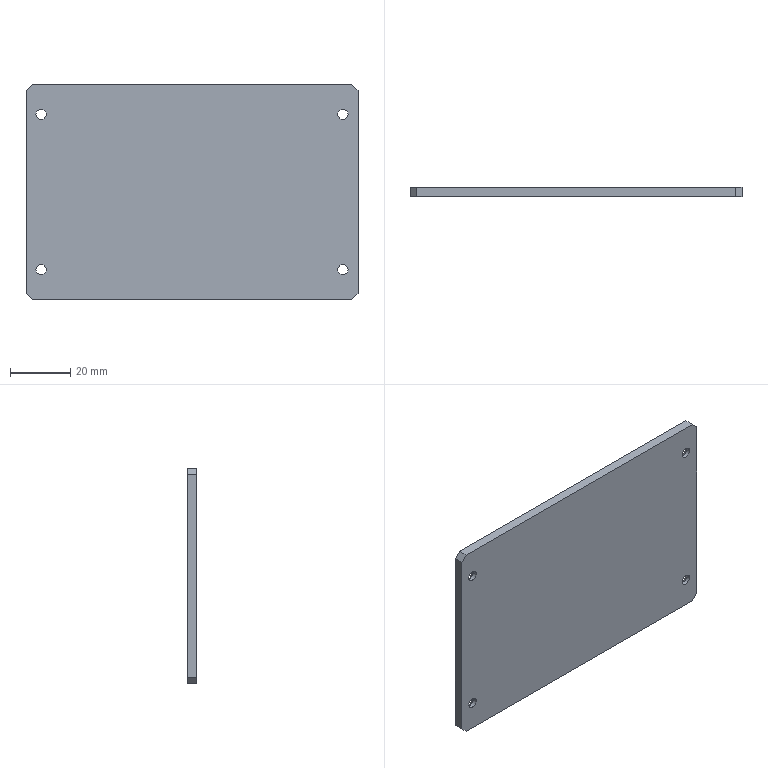Component | SolidWorks | 170423A4-SafetyPowerProbeFixingPlate5-1 | 1 solid | 26 faces | box 110 x 3 x 71.5 mm | volume 23384 mm3 | plane 10 | cone 8 | cylinder 8 | commonest cylinder face diameters 3.4 x8
build123d program:
from build123d import *

# Parameters (mm, degrees)
SKETCH1_W                                            = 110
SKETCH1_H                                            = 71.5
BOSS_EXTRUDE1_DEPTH                                  = 3
CHAMFER1_SIZE                                        = 2
M3_HEXAGONAL_COUNTERSUNK_HOLE_FOR_COUNTE_D           = 3.4
M3_HEXAGONAL_COUNTERSUNK_HOLE_FOR_COUNTE_DEPTH       = 8.5
M3_HEXAGONAL_COUNTERSUNK_HOLE_FOR_COUNTE_CSINK_D     = 6.72
M3_HEXAGONAL_COUNTERSUNK_HOLE_FOR_COUNTE_CSINK_ANGLE = 90
M3_HEXAGONAL_COUNTERSUNK_HOLE_FOR_COUNTE_TIP         = 1.021


with BuildPart() as part:
    # Sketch1 → Boss-Extrude1 (new body)
    with BuildSketch(Plane.XY):
        Rectangle(SKETCH1_W, SKETCH1_H)
    extrude(amount=BOSS_EXTRUDE1_DEPTH)

    # Chamfer1
    chamfer1_edges = [part.edges().sort_by_distance(p)[0] for p in [
        (55, -35.75, 1.5),
        (-55, -35.75, 1.5),
        (-55, 35.75, 1.5),
        (55, 35.75, 1.5),
    ]]
    chamfer(chamfer1_edges, length=CHAMFER1_SIZE)

    # M3 Hexagonal Countersunk Hole for Counte
    with Locations(Plane.XY.offset(3)):
        with Locations((50, -25.75), (50, 25.75), (-50, -25.75), (-50, 25.75)):
            CounterSinkHole(M3_HEXAGONAL_COUNTERSUNK_HOLE_FOR_COUNTE_D / 2, M3_HEXAGONAL_COUNTERSUNK_HOLE_FOR_COUNTE_CSINK_D / 2, depth=M3_HEXAGONAL_COUNTERSUNK_HOLE_FOR_COUNTE_DEPTH, counter_sink_angle=M3_HEXAGONAL_COUNTERSUNK_HOLE_FOR_COUNTE_CSINK_ANGLE)
            with Locations((0, 0, -(M3_HEXAGONAL_COUNTERSUNK_HOLE_FOR_COUNTE_DEPTH + M3_HEXAGONAL_COUNTERSUNK_HOLE_FOR_COUNTE_TIP / 2))):  # 118° drill point
                Cone(0, M3_HEXAGONAL_COUNTERSUNK_HOLE_FOR_COUNTE_D / 2, M3_HEXAGONAL_COUNTERSUNK_HOLE_FOR_COUNTE_TIP, mode=Mode.SUBTRACT)


solid = part.part

# Placed as in the assembly
solid = solid.moved(Location((28.687, 39.389, -37.824), (-90, 0, 0)))
STEP:
#1=COLOUR_RGB('',0.7922,0.8196,0.9333);
#2=FILL_AREA_STYLE_COLOUR('',#1);
#3=FILL_AREA_STYLE('',(#2));
#4=SURFACE_STYLE_FILL_AREA(#3);
#5=SURFACE_SIDE_STYLE('',(#4));
#6=SURFACE_STYLE_USAGE(.BOTH.,#5);
#7=PRESENTATION_STYLE_ASSIGNMENT((#6));
#8=CARTESIAN_POINT('',(-0.7722,1.604,-2.503));
#9=VERTEX_POINT('',#8);
#10=CARTESIAN_POINT('',(-0.906,1.604,-2.503));
#11=VERTEX_POINT('',#10);
#12=CARTESIAN_POINT('',(-0.8391,1.604,-2.503));
#13=DIRECTION('',(-0.,1.,-0.));
#14=DIRECTION('',(-1.,0.,0.));
#15=AXIS2_PLACEMENT_3D('',#12,#13,#14);
#16=CIRCLE('',#15,0.06693);
#17=EDGE_CURVE('',#9,#11,#16,.T.);
#18=ORIENTED_EDGE('',*,*,#17,.F.);
#19=CARTESIAN_POINT('',(-0.7068,1.669,-2.503));
#20=VERTEX_POINT('',#19);
#21=CARTESIAN_POINT('',(-0.7068,1.669,-2.503));
#22=DIRECTION('',(0.7071,0.7071,-0.));
#23=VECTOR('',#22,39.37);
#24=LINE('',#21,#23);
#25=EDGE_CURVE('',#9,#20,#24,.T.);
#26=ORIENTED_EDGE('',*,*,#25,.T.);
#27=CARTESIAN_POINT('',(-0.9714,1.669,-2.503));
#28=VERTEX_POINT('',#27);
#29=CARTESIAN_POINT('',(-0.8391,1.669,-2.503));
#30=DIRECTION('',(-0.,1.,-0.));
#31=DIRECTION('',(-1.,0.,0.));
#32=AXIS2_PLACEMENT_3D('',#29,#30,#31);
#33=CIRCLE('',#32,0.1323);
#34=EDGE_CURVE('',#20,#28,#33,.T.);
#35=ORIENTED_EDGE('',*,*,#34,.T.);
#36=CARTESIAN_POINT('',(-0.9714,1.669,-2.503));
#37=DIRECTION('',(-0.7071,0.7071,-0.));
#38=VECTOR('',#37,39.37);
#39=LINE('',#36,#38);
#40=EDGE_CURVE('',#11,#28,#39,.T.);
#41=ORIENTED_EDGE('',*,*,#40,.F.);
#42=EDGE_LOOP('',(#18,#26,#35,#41));
#43=FACE_OUTER_BOUND('',#42,.T.);
#44=CARTESIAN_POINT('',(-0.8391,1.669,-2.503));
#45=DIRECTION('',(-0.,1.,-0.));
#46=DIRECTION('',(-1.,0.,0.));
#47=AXIS2_PLACEMENT_3D('',#44,#45,#46);
#48=CONICAL_SURFACE('',#47,0.1323,0.7854);
#49=ADVANCED_FACE('',(#43),#48,.F.);
#50=CARTESIAN_POINT('',(-0.7722,1.551,-2.503));
#51=VERTEX_POINT('',#50);
#52=CARTESIAN_POINT('',(-0.906,1.551,-2.503));
#53=VERTEX_POINT('',#52);
#54=CARTESIAN_POINT('',(-0.8391,1.551,-2.503));
#55=DIRECTION('',(-0.,1.,-0.));
#56=DIRECTION('',(-1.,0.,0.));
#57=AXIS2_PLACEMENT_3D('',#54,#55,#56);
#58=CIRCLE('',#57,0.06693);
#59=EDGE_CURVE('',#51,#53,#58,.T.);
#60=ORIENTED_EDGE('',*,*,#59,.F.);
#61=CARTESIAN_POINT('',(-0.7722,1.669,-2.503));
#62=DIRECTION('',(-0.,1.,-0.));
#63=VECTOR('',#62,39.37);
#64=LINE('',#61,#63);
#65=EDGE_CURVE('',#51,#9,#64,.T.);
#66=ORIENTED_EDGE('',*,*,#65,.T.);
#67=ORIENTED_EDGE('',*,*,#17,.T.);
#68=CARTESIAN_POINT('',(-0.906,1.669,-2.503));
#69=DIRECTION('',(-0.,1.,-0.));
#70=VECTOR('',#69,39.37);
#71=LINE('',#68,#70);
#72=EDGE_CURVE('',#53,#11,#71,.T.);
#73=ORIENTED_EDGE('',*,*,#72,.F.);
#74=EDGE_LOOP('',(#60,#66,#67,#73));
#75=FACE_OUTER_BOUND('',#74,.T.);
#76=CARTESIAN_POINT('',(-0.8391,1.669,-2.503));
#77=DIRECTION('',(-0.,1.,-0.));
#78=DIRECTION('',(-1.,0.,0.));
#79=AXIS2_PLACEMENT_3D('',#76,#77,#78);
#80=CYLINDRICAL_SURFACE('',#79,0.06693);
#81=ADVANCED_FACE('',(#75),#80,.F.);
#82=CARTESIAN_POINT('',(-0.7722,1.604,-0.4753));
#83=VERTEX_POINT('',#82);
#84=CARTESIAN_POINT('',(-0.906,1.604,-0.4753));
#85=VERTEX_POINT('',#84);
#86=CARTESIAN_POINT('',(-0.8391,1.604,-0.4753));
#87=DIRECTION('',(-0.,1.,-0.));
#88=DIRECTION('',(-1.,0.,0.));
#89=AXIS2_PLACEMENT_3D('',#86,#87,#88);
#90=CIRCLE('',#89,0.06693);
#91=EDGE_CURVE('',#83,#85,#90,.T.);
#92=ORIENTED_EDGE('',*,*,#91,.F.);
#93=CARTESIAN_POINT('',(-0.7068,1.669,-0.4753));
#94=VERTEX_POINT('',#93);
#95=CARTESIAN_POINT('',(-0.7068,1.669,-0.4753));
#96=DIRECTION('',(0.7071,0.7071,-0.));
#97=VECTOR('',#96,39.37);
#98=LINE('',#95,#97);
#99=EDGE_CURVE('',#83,#94,#98,.T.);
#100=ORIENTED_EDGE('',*,*,#99,.T.);
#101=CARTESIAN_POINT('',(-0.9714,1.669,-0.4753));
#102=VERTEX_POINT('',#101);
#103=CARTESIAN_POINT('',(-0.8391,1.669,-0.4753));
#104=DIRECTION('',(-0.,1.,-0.));
#105=DIRECTION('',(-1.,0.,0.));
#106=AXIS2_PLACEMENT_3D('',#103,#104,#105);
#107=CIRCLE('',#106,0.1323);
#108=EDGE_CURVE('',#94,#102,#107,.T.);
#109=ORIENTED_EDGE('',*,*,#108,.T.);
#110=CARTESIAN_POINT('',(-0.9714,1.669,-0.4753));
#111=DIRECTION('',(-0.7071,0.7071,-0.));
#112=VECTOR('',#111,39.37);
#113=LINE('',#110,#112);
#114=EDGE_CURVE('',#85,#102,#113,.T.);
#115=ORIENTED_EDGE('',*,*,#114,.F.);
#116=EDGE_LOOP('',(#92,#100,#109,#115));
#117=FACE_OUTER_BOUND('',#116,.T.);
#118=CARTESIAN_POINT('',(-0.8391,1.669,-0.4753));
#119=DIRECTION('',(-0.,1.,-0.));
#120=DIRECTION('',(-1.,0.,0.));
#121=AXIS2_PLACEMENT_3D('',#118,#119,#120);
#122=CONICAL_SURFACE('',#121,0.1323,0.7854);
#123=ADVANCED_FACE('',(#117),#122,.F.);
#124=CARTESIAN_POINT('',(-0.7722,1.551,-0.4753));
#125=VERTEX_POINT('',#124);
#126=CARTESIAN_POINT('',(-0.906,1.551,-0.4753));
#127=VERTEX_POINT('',#126);
#128=CARTESIAN_POINT('',(-0.8391,1.551,-0.4753));
#129=DIRECTION('',(-0.,1.,-0.));
#130=DIRECTION('',(-1.,0.,0.));
#131=AXIS2_PLACEMENT_3D('',#128,#129,#130);
#132=CIRCLE('',#131,0.06693);
#133=EDGE_CURVE('',#125,#127,#132,.T.);
#134=ORIENTED_EDGE('',*,*,#133,.F.);
#135=CARTESIAN_POINT('',(-0.7722,1.669,-0.4753));
#136=DIRECTION('',(-0.,1.,-0.));
#137=VECTOR('',#136,39.37);
#138=LINE('',#135,#137);
#139=EDGE_CURVE('',#125,#83,#138,.T.);
#140=ORIENTED_EDGE('',*,*,#139,.T.);
#141=ORIENTED_EDGE('',*,*,#91,.T.);
#142=CARTESIAN_POINT('',(-0.906,1.669,-0.4753));
#143=DIRECTION('',(-0.,1.,-0.));
#144=VECTOR('',#143,39.37);
#145=LINE('',#142,#144);
#146=EDGE_CURVE('',#127,#85,#145,.T.);
#147=ORIENTED_EDGE('',*,*,#146,.F.);
#148=EDGE_LOOP('',(#134,#140,#141,#147));
#149=FACE_OUTER_BOUND('',#148,.T.);
#150=CARTESIAN_POINT('',(-0.8391,1.669,-0.4753));
#151=DIRECTION('',(-0.,1.,-0.));
#152=DIRECTION('',(-1.,0.,0.));
#153=AXIS2_PLACEMENT_3D('',#150,#151,#152);
#154=CYLINDRICAL_SURFACE('',#153,0.06693);
#155=ADVANCED_FACE('',(#149),#154,.F.);
#156=CARTESIAN_POINT('',(3.165,1.604,-2.503));
#157=VERTEX_POINT('',#156);
#158=CARTESIAN_POINT('',(3.031,1.604,-2.503));
#159=VERTEX_POINT('',#158);
#160=CARTESIAN_POINT('',(3.098,1.604,-2.503));
#161=DIRECTION('',(-0.,1.,-0.));
#162=DIRECTION('',(-1.,0.,0.));
#163=AXIS2_PLACEMENT_3D('',#160,#161,#162);
#164=CIRCLE('',#163,0.06693);
#165=EDGE_CURVE('',#157,#159,#164,.T.);
#166=ORIENTED_EDGE('',*,*,#165,.F.);
#167=CARTESIAN_POINT('',(3.23,1.669,-2.503));
#168=VERTEX_POINT('',#167);
#169=CARTESIAN_POINT('',(3.23,1.669,-2.503));
#170=DIRECTION('',(0.7071,0.7071,-0.));
#171=VECTOR('',#170,39.37);
#172=LINE('',#169,#171);
#173=EDGE_CURVE('',#157,#168,#172,.T.);
#174=ORIENTED_EDGE('',*,*,#173,.T.);
#175=CARTESIAN_POINT('',(2.966,1.669,-2.503));
#176=VERTEX_POINT('',#175);
#177=CARTESIAN_POINT('',(3.098,1.669,-2.503));
#178=DIRECTION('',(-0.,1.,-0.));
#179=DIRECTION('',(-1.,0.,0.));
#180=AXIS2_PLACEMENT_3D('',#177,#178,#179);
#181=CIRCLE('',#180,0.1323);
#182=EDGE_CURVE('',#168,#176,#181,.T.);
#183=ORIENTED_EDGE('',*,*,#182,.T.);
#184=CARTESIAN_POINT('',(2.966,1.669,-2.503));
#185=DIRECTION('',(-0.7071,0.7071,-0.));
#186=VECTOR('',#185,39.37);
#187=LINE('',#184,#186);
#188=EDGE_CURVE('',#159,#176,#187,.T.);
#189=ORIENTED_EDGE('',*,*,#188,.F.);
#190=EDGE_LOOP('',(#166,#174,#183,#189));
#191=FACE_OUTER_BOUND('',#190,.T.);
#192=CARTESIAN_POINT('',(3.098,1.669,-2.503));
#193=DIRECTION('',(-0.,1.,-0.));
#194=DIRECTION('',(-1.,0.,0.));
#195=AXIS2_PLACEMENT_3D('',#192,#193,#194);
#196=CONICAL_SURFACE('',#195,0.1323,0.7854);
#197=ADVANCED_FACE('',(#191),#196,.F.);
#198=CARTESIAN_POINT('',(3.165,1.551,-2.503));
#199=VERTEX_POINT('',#198);
#200=CARTESIAN_POINT('',(3.031,1.551,-2.503));
#201=VERTEX_POINT('',#200);
#202=CARTESIAN_POINT('',(3.098,1.551,-2.503));
#203=DIRECTION('',(-0.,1.,-0.));
#204=DIRECTION('',(-1.,0.,0.));
#205=AXIS2_PLACEMENT_3D('',#202,#203,#204);
#206=CIRCLE('',#205,0.06693);
#207=EDGE_CURVE('',#199,#201,#206,.T.);
#208=ORIENTED_EDGE('',*,*,#207,.F.);
#209=CARTESIAN_POINT('',(3.165,1.669,-2.503));
#210=DIRECTION('',(-0.,1.,-0.));
#211=VECTOR('',#210,39.37);
#212=LINE('',#209,#211);
#213=EDGE_CURVE('',#199,#157,#212,.T.);
#214=ORIENTED_EDGE('',*,*,#213,.T.);
#215=ORIENTED_EDGE('',*,*,#165,.T.);
#216=CARTESIAN_POINT('',(3.031,1.669,-2.503));
#217=DIRECTION('',(-0.,1.,-0.));
#218=VECTOR('',#217,39.37);
#219=LINE('',#216,#218);
#220=EDGE_CURVE('',#201,#159,#219,.T.);
#221=ORIENTED_EDGE('',*,*,#220,.F.);
#222=EDGE_LOOP('',(#208,#214,#215,#221));
#223=FACE_OUTER_BOUND('',#222,.T.);
#224=CARTESIAN_POINT('',(3.098,1.669,-2.503));
#225=DIRECTION('',(-0.,1.,-0.));
#226=DIRECTION('',(-1.,0.,0.));
#227=AXIS2_PLACEMENT_3D('',#224,#225,#226);
#228=CYLINDRICAL_SURFACE('',#227,0.06693);
#229=ADVANCED_FACE('',(#223),#228,.F.);
#230=CARTESIAN_POINT('',(3.165,1.604,-0.4753));
#231=VERTEX_POINT('',#230);
#232=CARTESIAN_POINT('',(3.031,1.604,-0.4753));
#233=VERTEX_POINT('',#232);
#234=CARTESIAN_POINT('',(3.098,1.604,-0.4753));
#235=DIRECTION('',(-0.,1.,-0.));
#236=DIRECTION('',(-1.,0.,0.));
#237=AXIS2_PLACEMENT_3D('',#234,#235,#236);
#238=CIRCLE('',#237,0.06693);
#239=EDGE_CURVE('',#231,#233,#238,.T.);
#240=ORIENTED_EDGE('',*,*,#239,.F.);
#241=CARTESIAN_POINT('',(3.23,1.669,-0.4753));
#242=VERTEX_POINT('',#241);
#243=CARTESIAN_POINT('',(3.23,1.669,-0.4753));
#244=DIRECTION('',(0.7071,0.7071,-0.));
#245=VECTOR('',#244,39.37);
#246=LINE('',#243,#245);
#247=EDGE_CURVE('',#231,#242,#246,.T.);
#248=ORIENTED_EDGE('',*,*,#247,.T.);
#249=CARTESIAN_POINT('',(2.966,1.669,-0.4753));
#250=VERTEX_POINT('',#249);
#251=CARTESIAN_POINT('',(3.098,1.669,-0.4753));
#252=DIRECTION('',(-0.,1.,-0.));
#253=DIRECTION('',(-1.,0.,0.));
#254=AXIS2_PLACEMENT_3D('',#251,#252,#253);
#255=CIRCLE('',#254,0.1323);
#256=EDGE_CURVE('',#242,#250,#255,.T.);
#257=ORIENTED_EDGE('',*,*,#256,.T.);
#258=CARTESIAN_POINT('',(2.966,1.669,-0.4753));
#259=DIRECTION('',(-0.7071,0.7071,-0.));
#260=VECTOR('',#259,39.37);
#261=LINE('',#258,#260);
#262=EDGE_CURVE('',#233,#250,#261,.T.);
#263=ORIENTED_EDGE('',*,*,#262,.F.);
#264=EDGE_LOOP('',(#240,#248,#257,#263));
#265=FACE_OUTER_BOUND('',#264,.T.);
#266=CARTESIAN_POINT('',(3.098,1.669,-0.4753));
#267=DIRECTION('',(-0.,1.,-0.));
#268=DIRECTION('',(-1.,0.,0.));
#269=AXIS2_PLACEMENT_3D('',#266,#267,#268);
#270=CONICAL_SURFACE('',#269,0.1323,0.7854);
#271=ADVANCED_FACE('',(#265),#270,.F.);
#272=CARTESIAN_POINT('',(3.165,1.551,-0.4753));
#273=VERTEX_POINT('',#272);
#274=CARTESIAN_POINT('',(3.031,1.551,-0.4753));
#275=VERTEX_POINT('',#274);
#276=CARTESIAN_POINT('',(3.098,1.551,-0.4753));
#277=DIRECTION('',(-0.,1.,-0.));
#278=DIRECTION('',(-1.,0.,0.));
#279=AXIS2_PLACEMENT_3D('',#276,#277,#278);
#280=CIRCLE('',#279,0.06693);
#281=EDGE_CURVE('',#273,#275,#280,.T.);
#282=ORIENTED_EDGE('',*,*,#281,.F.);
#283=CARTESIAN_POINT('',(3.165,1.669,-0.4753));
#284=DIRECTION('',(-0.,1.,-0.));
#285=VECTOR('',#284,39.37);
#286=LINE('',#283,#285);
#287=EDGE_CURVE('',#273,#231,#286,.T.);
#288=ORIENTED_EDGE('',*,*,#287,.T.);
#289=ORIENTED_EDGE('',*,*,#239,.T.);
#290=CARTESIAN_POINT('',(3.031,1.669,-0.4753));
#291=DIRECTION('',(-0.,1.,-0.));
#292=VECTOR('',#291,39.37);
#293=LINE('',#290,#292);
#294=EDGE_CURVE('',#275,#233,#293,.T.);
#295=ORIENTED_EDGE('',*,*,#294,.F.);
#296=EDGE_LOOP('',(#282,#288,#289,#295));
#297=FACE_OUTER_BOUND('',#296,.T.);
#298=CARTESIAN_POINT('',(3.098,1.669,-0.4753));
#299=DIRECTION('',(-0.,1.,-0.));
#300=DIRECTION('',(-1.,0.,0.));
#301=AXIS2_PLACEMENT_3D('',#298,#299,#300);
#302=CYLINDRICAL_SURFACE('',#301,0.06693);
#303=ADVANCED_FACE('',(#297),#302,.F.);
#304=CARTESIAN_POINT('',(-1.036,1.669,-2.818));
#305=VERTEX_POINT('',#304);
#306=CARTESIAN_POINT('',(-1.036,1.669,-0.1604));
#307=VERTEX_POINT('',#306);
#308=CARTESIAN_POINT('',(-1.036,1.669,-0.08165));
#309=DIRECTION('',(0.,0.,1.));
#310=VECTOR('',#309,39.37);
#311=LINE('',#308,#310);
#312=EDGE_CURVE('',#305,#307,#311,.T.);
#313=ORIENTED_EDGE('',*,*,#312,.F.);
#314=CARTESIAN_POINT('',(-1.036,1.551,-2.818));
#315=VERTEX_POINT('',#314);
#316=CARTESIAN_POINT('',(-1.036,1.669,-2.818));
#317=DIRECTION('',(0.,-1.,0.));
#318=VECTOR('',#317,39.37);
#319=LINE('',#316,#318);
#320=EDGE_CURVE('',#305,#315,#319,.T.);
#321=ORIENTED_EDGE('',*,*,#320,.T.);
#322=CARTESIAN_POINT('',(-1.036,1.551,-0.1604));
#323=VERTEX_POINT('',#322);
#324=CARTESIAN_POINT('',(-1.036,1.551,-0.08165));
#325=DIRECTION('',(0.,0.,1.));
#326=VECTOR('',#325,39.37);
#327=LINE('',#324,#326);
#328=EDGE_CURVE('',#315,#323,#327,.T.);
#329=ORIENTED_EDGE('',*,*,#328,.T.);
#330=CARTESIAN_POINT('',(-1.036,1.669,-0.1604));
#331=DIRECTION('',(-0.,1.,-0.));
#332=VECTOR('',#331,39.37);
#333=LINE('',#330,#332);
#334=EDGE_CURVE('',#323,#307,#333,.T.);
#335=ORIENTED_EDGE('',*,*,#334,.T.);
#336=EDGE_LOOP('',(#313,#321,#329,#335));
#337=FACE_OUTER_BOUND('',#336,.T.);
#338=CARTESIAN_POINT('',(-1.036,1.669,-0.08165));
#339=DIRECTION('',(1.,0.,-0.));
#340=DIRECTION('',(-0.,-0.,-1.));
#341=AXIS2_PLACEMENT_3D('',#338,#339,#340);
#342=PLANE('',#341);
#343=ADVANCED_FACE('',(#337),#342,.F.);
#344=CARTESIAN_POINT('',(-0.9572,1.669,-0.08165));
#345=VERTEX_POINT('',#344);
#346=CARTESIAN_POINT('',(3.216,1.669,-0.08165));
#347=VERTEX_POINT('',#346);
#348=CARTESIAN_POINT('',(3.295,1.669,-0.08165));
#349=DIRECTION('',(1.,0.,0.));
#350=VECTOR('',#349,39.37);
#351=LINE('',#348,#350);
#352=EDGE_CURVE('',#345,#347,#351,.T.);
#353=ORIENTED_EDGE('',*,*,#352,.F.);
#354=CARTESIAN_POINT('',(-0.9572,1.551,-0.08165));
#355=VERTEX_POINT('',#354);
#356=CARTESIAN_POINT('',(-0.9572,1.669,-0.08165));
#357=DIRECTION('',(0.,-1.,0.));
#358=VECTOR('',#357,39.37);
#359=LINE('',#356,#358);
#360=EDGE_CURVE('',#345,#355,#359,.T.);
#361=ORIENTED_EDGE('',*,*,#360,.T.);
#362=CARTESIAN_POINT('',(3.216,1.551,-0.08165));
#363=VERTEX_POINT('',#362);
#364=CARTESIAN_POINT('',(3.295,1.551,-0.08165));
#365=DIRECTION('',(1.,0.,0.));
#366=VECTOR('',#365,39.37);
#367=LINE('',#364,#366);
#368=EDGE_CURVE('',#355,#363,#367,.T.);
#369=ORIENTED_EDGE('',*,*,#368,.T.);
#370=CARTESIAN_POINT('',(3.216,1.669,-0.08165));
#371=DIRECTION('',(-0.,1.,-0.));
#372=VECTOR('',#371,39.37);
#373=LINE('',#370,#372);
#374=EDGE_CURVE('',#363,#347,#373,.T.);
#375=ORIENTED_EDGE('',*,*,#374,.T.);
#376=EDGE_LOOP('',(#353,#361,#369,#375));
#377=FACE_OUTER_BOUND('',#376,.T.);
#378=CARTESIAN_POINT('',(3.295,1.669,-0.08165));
#379=DIRECTION('',(-0.,-0.,-1.));
#380=DIRECTION('',(0.,-1.,0.));
#381=AXIS2_PLACEMENT_3D('',#378,#379,#380);
#382=PLANE('',#381);
#383=ADVANCED_FACE('',(#377),#382,.F.);
#384=CARTESIAN_POINT('',(3.295,1.551,-0.1604));
#385=VERTEX_POINT('',#384);
#386=CARTESIAN_POINT('',(3.295,1.551,-2.818));
#387=VERTEX_POINT('',#386);
#388=CARTESIAN_POINT('',(3.295,1.551,-0.08165));
#389=DIRECTION('',(-0.,-0.,-1.));
#390=VECTOR('',#389,39.37);
#391=LINE('',#388,#390);
#392=EDGE_CURVE('',#385,#387,#391,.T.);
#393=ORIENTED_EDGE('',*,*,#392,.T.);
#394=CARTESIAN_POINT('',(3.295,1.669,-2.818));
#395=VERTEX_POINT('',#394);
#396=CARTESIAN_POINT('',(3.295,1.669,-2.818));
#397=DIRECTION('',(-0.,1.,-0.));
#398=VECTOR('',#397,39.37);
#399=LINE('',#396,#398);
#400=EDGE_CURVE('',#387,#395,#399,.T.);
#401=ORIENTED_EDGE('',*,*,#400,.T.);
#402=CARTESIAN_POINT('',(3.295,1.669,-0.1604));
#403=VERTEX_POINT('',#402);
#404=CARTESIAN_POINT('',(3.295,1.669,-0.08165));
#405=DIRECTION('',(-0.,-0.,-1.));
#406=VECTOR('',#405,39.37);
#407=LINE('',#404,#406);
#408=EDGE_CURVE('',#403,#395,#407,.T.);
#409=ORIENTED_EDGE('',*,*,#408,.F.);
#410=CARTESIAN_POINT('',(3.295,1.669,-0.1604));
#411=DIRECTION('',(0.,-1.,0.));
#412=VECTOR('',#411,39.37);
#413=LINE('',#410,#412);
#414=EDGE_CURVE('',#403,#385,#413,.T.);
#415=ORIENTED_EDGE('',*,*,#414,.T.);
#416=EDGE_LOOP('',(#393,#401,#409,#415));
#417=FACE_OUTER_BOUND('',#416,.T.);
#418=CARTESIAN_POINT('',(3.295,1.669,-0.08165));
#419=DIRECTION('',(-1.,-0.,0.));
#420=DIRECTION('',(0.,0.,1.));
#421=AXIS2_PLACEMENT_3D('',#418,#419,#420);
#422=PLANE('',#421);
#423=ADVANCED_FACE('',(#417),#422,.F.);
#424=CARTESIAN_POINT('',(3.216,1.551,-2.897));
#425=VERTEX_POINT('',#424);
#426=CARTESIAN_POINT('',(-0.9572,1.551,-2.897));
#427=VERTEX_POINT('',#426);
#428=CARTESIAN_POINT('',(3.295,1.551,-2.897));
#429=DIRECTION('',(-1.,-0.,-0.));
#430=VECTOR('',#429,39.37);
#431=LINE('',#428,#430);
#432=EDGE_CURVE('',#425,#427,#431,.T.);
#433=ORIENTED_EDGE('',*,*,#432,.T.);
#434=CARTESIAN_POINT('',(-0.9572,1.669,-2.897));
#435=VERTEX_POINT('',#434);
#436=CARTESIAN_POINT('',(-0.9572,1.669,-2.897));
#437=DIRECTION('',(-0.,1.,-0.));
#438=VECTOR('',#437,39.37);
#439=LINE('',#436,#438);
#440=EDGE_CURVE('',#427,#435,#439,.T.);
#441=ORIENTED_EDGE('',*,*,#440,.T.);
#442=CARTESIAN_POINT('',(3.216,1.669,-2.897));
#443=VERTEX_POINT('',#442);
#444=CARTESIAN_POINT('',(3.295,1.669,-2.897));
#445=DIRECTION('',(-1.,-0.,-0.));
#446=VECTOR('',#445,39.37);
#447=LINE('',#444,#446);
#448=EDGE_CURVE('',#443,#435,#447,.T.);
#449=ORIENTED_EDGE('',*,*,#448,.F.);
#450=CARTESIAN_POINT('',(3.216,1.669,-2.897));
#451=DIRECTION('',(0.,-1.,0.));
#452=VECTOR('',#451,39.37);
#453=LINE('',#450,#452);
#454=EDGE_CURVE('',#443,#425,#453,.T.);
#455=ORIENTED_EDGE('',*,*,#454,.T.);
#456=EDGE_LOOP('',(#433,#441,#449,#455));
#457=FACE_OUTER_BOUND('',#456,.T.);
#458=CARTESIAN_POINT('',(3.295,1.669,-2.897));
#459=DIRECTION('',(0.,0.,1.));
#460=DIRECTION('',(-0.,1.,-0.));
#461=AXIS2_PLACEMENT_3D('',#458,#459,#460);
#462=PLANE('',#461);
#463=ADVANCED_FACE('',(#457),#462,.F.);
#464=CARTESIAN_POINT('',(-0.8391,1.669,-2.503));
#465=DIRECTION('',(-0.,1.,-0.));
#466=DIRECTION('',(-1.,0.,0.));
#467=AXIS2_PLACEMENT_3D('',#464,#465,#466);
#468=CIRCLE('',#467,0.1323);
#469=EDGE_CURVE('',#28,#20,#468,.T.);
#470=ORIENTED_EDGE('',*,*,#469,.F.);
#471=ORIENTED_EDGE('',*,*,#34,.F.);
#472=EDGE_LOOP('',(#470,#471));
#473=FACE_BOUND('',#472,.T.);
#474=CARTESIAN_POINT('',(-0.8391,1.669,-0.4753));
#475=DIRECTION('',(-0.,1.,-0.));
#476=DIRECTION('',(-1.,0.,0.));
#477=AXIS2_PLACEMENT_3D('',#474,#475,#476);
#478=CIRCLE('',#477,0.1323);
#479=EDGE_CURVE('',#102,#94,#478,.T.);
#480=ORIENTED_EDGE('',*,*,#479,.F.);
#481=ORIENTED_EDGE('',*,*,#108,.F.);
#482=EDGE_LOOP('',(#480,#481));
#483=FACE_BOUND('',#482,.T.);
#484=CARTESIAN_POINT('',(3.098,1.669,-2.503));
#485=DIRECTION('',(-0.,1.,-0.));
#486=DIRECTION('',(-1.,0.,0.));
#487=AXIS2_PLACEMENT_3D('',#484,#485,#486);
#488=CIRCLE('',#487,0.1323);
#489=EDGE_CURVE('',#176,#168,#488,.T.);
#490=ORIENTED_EDGE('',*,*,#489,.F.);
#491=ORIENTED_EDGE('',*,*,#182,.F.);
#492=EDGE_LOOP('',(#490,#491));
#493=FACE_BOUND('',#492,.T.);
#494=CARTESIAN_POINT('',(3.098,1.669,-0.4753));
#495=DIRECTION('',(-0.,1.,-0.));
#496=DIRECTION('',(-1.,0.,0.));
#497=AXIS2_PLACEMENT_3D('',#494,#495,#496);
#498=CIRCLE('',#497,0.1323);
#499=EDGE_CURVE('',#250,#242,#498,.T.);
#500=ORIENTED_EDGE('',*,*,#499,.F.);
#501=ORIENTED_EDGE('',*,*,#256,.F.);
#502=EDGE_LOOP('',(#500,#501));
#503=FACE_BOUND('',#502,.T.);
#504=ORIENTED_EDGE('',*,*,#448,.T.);
#505=CARTESIAN_POINT('',(-0.6177,1.669,-3.236));
#506=DIRECTION('',(-0.7071,0.,0.7071));
#507=VECTOR('',#506,39.37);
#508=LINE('',#505,#507);
#509=EDGE_CURVE('',#435,#305,#508,.T.);
#510=ORIENTED_EDGE('',*,*,#509,.T.);
#511=ORIENTED_EDGE('',*,*,#312,.T.);
#512=CARTESIAN_POINT('',(-0.6177,1.669,0.2579));
#513=DIRECTION('',(0.7071,0.,0.7071));
#514=VECTOR('',#513,39.37);
#515=LINE('',#512,#514);
#516=EDGE_CURVE('',#307,#345,#515,.T.);
#517=ORIENTED_EDGE('',*,*,#516,.T.);
#518=ORIENTED_EDGE('',*,*,#352,.T.);
#519=CARTESIAN_POINT('',(2.876,1.669,0.2579));
#520=DIRECTION('',(0.7071,-0.,-0.7071));
#521=VECTOR('',#520,39.37);
#522=LINE('',#519,#521);
#523=EDGE_CURVE('',#347,#403,#522,.T.);
#524=ORIENTED_EDGE('',*,*,#523,.T.);
#525=ORIENTED_EDGE('',*,*,#408,.T.);
#526=CARTESIAN_POINT('',(2.876,1.669,-3.236));
#527=DIRECTION('',(-0.7071,-0.,-0.7071));
#528=VECTOR('',#527,39.37);
#529=LINE('',#526,#528);
#530=EDGE_CURVE('',#395,#443,#529,.T.);
#531=ORIENTED_EDGE('',*,*,#530,.T.);
#532=EDGE_LOOP('',(#504,#510,#511,#517,#518,#524,#525,#531));
#533=FACE_OUTER_BOUND('',#532,.T.);
#534=CARTESIAN_POINT('',(1.129,1.669,-1.489));
#535=DIRECTION('',(0.,1.,-0.));
#536=DIRECTION('',(-1.,-0.,-0.));
#537=AXIS2_PLACEMENT_3D('',#534,#535,#536);
#538=PLANE('',#537);
#539=ADVANCED_FACE('',(#473,#483,#493,#503,#533),#538,.T.);
#540=CARTESIAN_POINT('',(-0.8391,1.551,-2.503));
#541=DIRECTION('',(-0.,1.,-0.));
#542=DIRECTION('',(-1.,0.,0.));
#543=AXIS2_PLACEMENT_3D('',#540,#541,#542);
#544=CIRCLE('',#543,0.06693);
#545=EDGE_CURVE('',#53,#51,#544,.T.);
#546=ORIENTED_EDGE('',*,*,#545,.T.);
#547=ORIENTED_EDGE('',*,*,#59,.T.);
#548=EDGE_LOOP('',(#546,#547));
#549=FACE_BOUND('',#548,.T.);
#550=CARTESIAN_POINT('',(-0.8391,1.551,-0.4753));
#551=DIRECTION('',(-0.,1.,-0.));
#552=DIRECTION('',(-1.,0.,0.));
#553=AXIS2_PLACEMENT_3D('',#550,#551,#552);
#554=CIRCLE('',#553,0.06693);
#555=EDGE_CURVE('',#127,#125,#554,.T.);
#556=ORIENTED_EDGE('',*,*,#555,.T.);
#557=ORIENTED_EDGE('',*,*,#133,.T.);
#558=EDGE_LOOP('',(#556,#557));
#559=FACE_BOUND('',#558,.T.);
#560=CARTESIAN_POINT('',(3.098,1.551,-2.503));
#561=DIRECTION('',(-0.,1.,-0.));
#562=DIRECTION('',(-1.,0.,0.));
#563=AXIS2_PLACEMENT_3D('',#560,#561,#562);
#564=CIRCLE('',#563,0.06693);
#565=EDGE_CURVE('',#201,#199,#564,.T.);
#566=ORIENTED_EDGE('',*,*,#565,.T.);
#567=ORIENTED_EDGE('',*,*,#207,.T.);
#568=EDGE_LOOP('',(#566,#567));
#569=FACE_BOUND('',#568,.T.);
#570=CARTESIAN_POINT('',(3.098,1.551,-0.4753));
#571=DIRECTION('',(-0.,1.,-0.));
#572=DIRECTION('',(-1.,0.,0.));
#573=AXIS2_PLACEMENT_3D('',#570,#571,#572);
#574=CIRCLE('',#573,0.06693);
#575=EDGE_CURVE('',#275,#273,#574,.T.);
#576=ORIENTED_EDGE('',*,*,#575,.T.);
#577=ORIENTED_EDGE('',*,*,#281,.T.);
#578=EDGE_LOOP('',(#576,#577));
#579=FACE_BOUND('',#578,.T.);
#580=ORIENTED_EDGE('',*,*,#328,.F.);
#581=CARTESIAN_POINT('',(-1.036,1.551,-2.818));
#582=DIRECTION('',(0.7071,-0.,-0.7071));
#583=VECTOR('',#582,39.37);
#584=LINE('',#581,#583);
#585=EDGE_CURVE('',#315,#427,#584,.T.);
#586=ORIENTED_EDGE('',*,*,#585,.T.);
#587=ORIENTED_EDGE('',*,*,#432,.F.);
#588=CARTESIAN_POINT('',(3.216,1.551,-2.897));
#589=DIRECTION('',(0.7071,0.,0.7071));
#590=VECTOR('',#589,39.37);
#591=LINE('',#588,#590);
#592=EDGE_CURVE('',#425,#387,#591,.T.);
#593=ORIENTED_EDGE('',*,*,#592,.T.);
#594=ORIENTED_EDGE('',*,*,#392,.F.);
#595=CARTESIAN_POINT('',(3.295,1.551,-0.1604));
#596=DIRECTION('',(-0.7071,0.,0.7071));
#597=VECTOR('',#596,39.37);
#598=LINE('',#595,#597);
#599=EDGE_CURVE('',#385,#363,#598,.T.);
#600=ORIENTED_EDGE('',*,*,#599,.T.);
#601=ORIENTED_EDGE('',*,*,#368,.F.);
#602=CARTESIAN_POINT('',(-0.9572,1.551,-0.08165));
#603=DIRECTION('',(-0.7071,-0.,-0.7071));
#604=VECTOR('',#603,39.37);
#605=LINE('',#602,#604);
#606=EDGE_CURVE('',#355,#323,#605,.T.);
#607=ORIENTED_EDGE('',*,*,#606,.T.);
#608=EDGE_LOOP('',(#580,#586,#587,#593,#594,#600,#601,#607));
#609=FACE_OUTER_BOUND('',#608,.T.);
#610=CARTESIAN_POINT('',(1.129,1.551,-1.489));
#611=DIRECTION('',(0.,1.,-0.));
#612=DIRECTION('',(-1.,-0.,-0.));
#613=AXIS2_PLACEMENT_3D('',#610,#611,#612);
#614=PLANE('',#613);
#615=ADVANCED_FACE('',(#549,#559,#569,#579,#609),#614,.F.);
#616=ORIENTED_EDGE('',*,*,#509,.F.);
#617=ORIENTED_EDGE('',*,*,#440,.F.);
#618=ORIENTED_EDGE('',*,*,#585,.F.);
#619=ORIENTED_EDGE('',*,*,#320,.F.);
#620=EDGE_LOOP('',(#616,#617,#618,#619));
#621=FACE_OUTER_BOUND('',#620,.T.);
#622=CARTESIAN_POINT('',(-1.036,1.669,-2.818));
#623=DIRECTION('',(0.7071,0.,0.7071));
#624=DIRECTION('',(0.,-1.,0.));
#625=AXIS2_PLACEMENT_3D('',#622,#623,#624);
#626=PLANE('',#625);
#627=ADVANCED_FACE('',(#621),#626,.F.);
#628=ORIENTED_EDGE('',*,*,#516,.F.);
#629=ORIENTED_EDGE('',*,*,#334,.F.);
#630=ORIENTED_EDGE('',*,*,#606,.F.);
#631=ORIENTED_EDGE('',*,*,#360,.F.);
#632=EDGE_LOOP('',(#628,#629,#630,#631));
#633=FACE_OUTER_BOUND('',#632,.T.);
#634=CARTESIAN_POINT('',(-0.9572,1.669,-0.08165));
#635=DIRECTION('',(0.7071,-0.,-0.7071));
#636=DIRECTION('',(0.,-1.,0.));
#637=AXIS2_PLACEMENT_3D('',#634,#635,#636);
#638=PLANE('',#637);
#639=ADVANCED_FACE('',(#633),#638,.F.);
#640=ORIENTED_EDGE('',*,*,#530,.F.);
#641=ORIENTED_EDGE('',*,*,#400,.F.);
#642=ORIENTED_EDGE('',*,*,#592,.F.);
#643=ORIENTED_EDGE('',*,*,#454,.F.);
#644=EDGE_LOOP('',(#640,#641,#642,#643));
#645=FACE_OUTER_BOUND('',#644,.T.);
#646=CARTESIAN_POINT('',(3.216,1.669,-2.897));
#647=DIRECTION('',(-0.7071,0.,0.7071));
#648=DIRECTION('',(0.,-1.,0.));
#649=AXIS2_PLACEMENT_3D('',#646,#647,#648);
#650=PLANE('',#649);
#651=ADVANCED_FACE('',(#645),#650,.F.);
#652=ORIENTED_EDGE('',*,*,#523,.F.);
#653=ORIENTED_EDGE('',*,*,#374,.F.);
#654=ORIENTED_EDGE('',*,*,#599,.F.);
#655=ORIENTED_EDGE('',*,*,#414,.F.);
#656=EDGE_LOOP('',(#652,#653,#654,#655));
#657=FACE_OUTER_BOUND('',#656,.T.);
#658=CARTESIAN_POINT('',(3.295,1.669,-0.1604));
#659=DIRECTION('',(-0.7071,-0.,-0.7071));
#660=DIRECTION('',(0.,-1.,0.));
#661=AXIS2_PLACEMENT_3D('',#658,#659,#660);
#662=PLANE('',#661);
#663=ADVANCED_FACE('',(#657),#662,.F.);
#664=ORIENTED_EDGE('',*,*,#287,.F.);
#665=ORIENTED_EDGE('',*,*,#575,.F.);
#666=ORIENTED_EDGE('',*,*,#294,.T.);
#667=CARTESIAN_POINT('',(3.098,1.604,-0.4753));
#668=DIRECTION('',(-0.,1.,-0.));
#669=DIRECTION('',(-1.,0.,0.));
#670=AXIS2_PLACEMENT_3D('',#667,#668,#669);
#671=CIRCLE('',#670,0.06693);
#672=EDGE_CURVE('',#233,#231,#671,.T.);
#673=ORIENTED_EDGE('',*,*,#672,.T.);
#674=EDGE_LOOP('',(#664,#665,#666,#673));
#675=FACE_OUTER_BOUND('',#674,.T.);
#676=CARTESIAN_POINT('',(3.098,1.669,-0.4753));
#677=DIRECTION('',(-0.,1.,-0.));
#678=DIRECTION('',(-1.,0.,0.));
#679=AXIS2_PLACEMENT_3D('',#676,#677,#678);
#680=CYLINDRICAL_SURFACE('',#679,0.06693);
#681=ADVANCED_FACE('',(#675),#680,.F.);
#682=ORIENTED_EDGE('',*,*,#247,.F.);
#683=ORIENTED_EDGE('',*,*,#672,.F.);
#684=ORIENTED_EDGE('',*,*,#262,.T.);
#685=ORIENTED_EDGE('',*,*,#499,.T.);
#686=EDGE_LOOP('',(#682,#683,#684,#685));
#687=FACE_OUTER_BOUND('',#686,.T.);
#688=CARTESIAN_POINT('',(3.098,1.669,-0.4753));
#689=DIRECTION('',(-0.,1.,-0.));
#690=DIRECTION('',(-1.,0.,0.));
#691=AXIS2_PLACEMENT_3D('',#688,#689,#690);
#692=CONICAL_SURFACE('',#691,0.1323,0.7854);
#693=ADVANCED_FACE('',(#687),#692,.F.);
#694=ORIENTED_EDGE('',*,*,#213,.F.);
#695=ORIENTED_EDGE('',*,*,#565,.F.);
#696=ORIENTED_EDGE('',*,*,#220,.T.);
#697=CARTESIAN_POINT('',(3.098,1.604,-2.503));
#698=DIRECTION('',(-0.,1.,-0.));
#699=DIRECTION('',(-1.,0.,0.));
#700=AXIS2_PLACEMENT_3D('',#697,#698,#699);
#701=CIRCLE('',#700,0.06693);
#702=EDGE_CURVE('',#159,#157,#701,.T.);
#703=ORIENTED_EDGE('',*,*,#702,.T.);
#704=EDGE_LOOP('',(#694,#695,#696,#703));
#705=FACE_OUTER_BOUND('',#704,.T.);
#706=CARTESIAN_POINT('',(3.098,1.669,-2.503));
#707=DIRECTION('',(-0.,1.,-0.));
#708=DIRECTION('',(-1.,0.,0.));
#709=AXIS2_PLACEMENT_3D('',#706,#707,#708);
#710=CYLINDRICAL_SURFACE('',#709,0.06693);
#711=ADVANCED_FACE('',(#705),#710,.F.);
#712=ORIENTED_EDGE('',*,*,#173,.F.);
#713=ORIENTED_EDGE('',*,*,#702,.F.);
#714=ORIENTED_EDGE('',*,*,#188,.T.);
#715=ORIENTED_EDGE('',*,*,#489,.T.);
#716=EDGE_LOOP('',(#712,#713,#714,#715));
#717=FACE_OUTER_BOUND('',#716,.T.);
#718=CARTESIAN_POINT('',(3.098,1.669,-2.503));
#719=DIRECTION('',(-0.,1.,-0.));
#720=DIRECTION('',(-1.,0.,0.));
#721=AXIS2_PLACEMENT_3D('',#718,#719,#720);
#722=CONICAL_SURFACE('',#721,0.1323,0.7854);
#723=ADVANCED_FACE('',(#717),#722,.F.);
#724=ORIENTED_EDGE('',*,*,#139,.F.);
#725=ORIENTED_EDGE('',*,*,#555,.F.);
#726=ORIENTED_EDGE('',*,*,#146,.T.);
#727=CARTESIAN_POINT('',(-0.8391,1.604,-0.4753));
#728=DIRECTION('',(-0.,1.,-0.));
#729=DIRECTION('',(-1.,0.,0.));
#730=AXIS2_PLACEMENT_3D('',#727,#728,#729);
#731=CIRCLE('',#730,0.06693);
#732=EDGE_CURVE('',#85,#83,#731,.T.);
#733=ORIENTED_EDGE('',*,*,#732,.T.);
#734=EDGE_LOOP('',(#724,#725,#726,#733));
#735=FACE_OUTER_BOUND('',#734,.T.);
#736=CARTESIAN_POINT('',(-0.8391,1.669,-0.4753));
#737=DIRECTION('',(-0.,1.,-0.));
#738=DIRECTION('',(-1.,0.,0.));
#739=AXIS2_PLACEMENT_3D('',#736,#737,#738);
#740=CYLINDRICAL_SURFACE('',#739,0.06693);
#741=ADVANCED_FACE('',(#735),#740,.F.);
#742=ORIENTED_EDGE('',*,*,#99,.F.);
#743=ORIENTED_EDGE('',*,*,#732,.F.);
#744=ORIENTED_EDGE('',*,*,#114,.T.);
#745=ORIENTED_EDGE('',*,*,#479,.T.);
#746=EDGE_LOOP('',(#742,#743,#744,#745));
#747=FACE_OUTER_BOUND('',#746,.T.);
#748=CARTESIAN_POINT('',(-0.8391,1.669,-0.4753));
#749=DIRECTION('',(-0.,1.,-0.));
#750=DIRECTION('',(-1.,0.,0.));
#751=AXIS2_PLACEMENT_3D('',#748,#749,#750);
#752=CONICAL_SURFACE('',#751,0.1323,0.7854);
#753=ADVANCED_FACE('',(#747),#752,.F.);
#754=ORIENTED_EDGE('',*,*,#65,.F.);
#755=ORIENTED_EDGE('',*,*,#545,.F.);
#756=ORIENTED_EDGE('',*,*,#72,.T.);
#757=CARTESIAN_POINT('',(-0.8391,1.604,-2.503));
#758=DIRECTION('',(-0.,1.,-0.));
#759=DIRECTION('',(-1.,0.,0.));
#760=AXIS2_PLACEMENT_3D('',#757,#758,#759);
#761=CIRCLE('',#760,0.06693);
#762=EDGE_CURVE('',#11,#9,#761,.T.);
#763=ORIENTED_EDGE('',*,*,#762,.T.);
#764=EDGE_LOOP('',(#754,#755,#756,#763));
#765=FACE_OUTER_BOUND('',#764,.T.);
#766=CARTESIAN_POINT('',(-0.8391,1.669,-2.503));
#767=DIRECTION('',(-0.,1.,-0.));
#768=DIRECTION('',(-1.,0.,0.));
#769=AXIS2_PLACEMENT_3D('',#766,#767,#768);
#770=CYLINDRICAL_SURFACE('',#769,0.06693);
#771=ADVANCED_FACE('',(#765),#770,.F.);
#772=ORIENTED_EDGE('',*,*,#25,.F.);
#773=ORIENTED_EDGE('',*,*,#762,.F.);
#774=ORIENTED_EDGE('',*,*,#40,.T.);
#775=ORIENTED_EDGE('',*,*,#469,.T.);
#776=EDGE_LOOP('',(#772,#773,#774,#775));
#777=FACE_OUTER_BOUND('',#776,.T.);
#778=CARTESIAN_POINT('',(-0.8391,1.669,-2.503));
#779=DIRECTION('',(-0.,1.,-0.));
#780=DIRECTION('',(-1.,0.,0.));
#781=AXIS2_PLACEMENT_3D('',#778,#779,#780);
#782=CONICAL_SURFACE('',#781,0.1323,0.7854);
#783=ADVANCED_FACE('',(#777),#782,.F.);
#784=CLOSED_SHELL('',(#49,#81,#123,#155,#197,#229,#271,#303,#343,#383,#423,#463,#539,#615,#627,#639,#651,#663,#681,#693,#711,#723,#741,#753,#771,#783));
#785=MANIFOLD_SOLID_BREP('',#784);
#786=STYLED_ITEM('',(#7),#785);
#787=(LENGTH_UNIT()NAMED_UNIT(*)SI_UNIT($,.METRE.));
#788=LENGTH_MEASURE_WITH_UNIT(LENGTH_MEASURE(0.0254),#787);
#789=DIMENSIONAL_EXPONENTS(1.,0.,0.,0.,0.,0.,0.);
#790=(CONVERSION_BASED_UNIT('',#788)LENGTH_UNIT()NAMED_UNIT(#789));
#791=UNCERTAINTY_MEASURE_WITH_UNIT(LENGTH_MEASURE(0.00001),#790,'','');
#792=(NAMED_UNIT(*)PLANE_ANGLE_UNIT()SI_UNIT($,.RADIAN.));
#793=(NAMED_UNIT(*)SI_UNIT($,.STERADIAN.)SOLID_ANGLE_UNIT());
#794=(GEOMETRIC_REPRESENTATION_CONTEXT(3)GLOBAL_UNCERTAINTY_ASSIGNED_CONTEXT((#791))GLOBAL_UNIT_ASSIGNED_CONTEXT((#790,#792,#793))REPRESENTATION_CONTEXT('',''));
#795=MECHANICAL_DESIGN_GEOMETRIC_PRESENTATION_REPRESENTATION('',(#786),#794);
#796=PRESENTATION_LAYER_ASSIGNMENT('','',(#786));
#797=CARTESIAN_POINT('',(0.,0.,0.));
#798=DIRECTION('',(0.,0.,1.));
#799=DIRECTION('',(1.,0.,0.));
#800=AXIS2_PLACEMENT_3D('',#797,#798,#799);
#801=(LENGTH_UNIT()NAMED_UNIT(*)SI_UNIT($,.METRE.));
#802=LENGTH_MEASURE_WITH_UNIT(LENGTH_MEASURE(0.0254),#801);
#803=DIMENSIONAL_EXPONENTS(1.,0.,0.,0.,0.,0.,0.);
#804=(CONVERSION_BASED_UNIT('',#802)LENGTH_UNIT()NAMED_UNIT(#803));
#805=UNCERTAINTY_MEASURE_WITH_UNIT(LENGTH_MEASURE(0.00001),#804,'','');
#806=(NAMED_UNIT(*)PLANE_ANGLE_UNIT()SI_UNIT($,.RADIAN.));
#807=(NAMED_UNIT(*)SI_UNIT($,.STERADIAN.)SOLID_ANGLE_UNIT());
#808=(GEOMETRIC_REPRESENTATION_CONTEXT(3)GLOBAL_UNCERTAINTY_ASSIGNED_CONTEXT((#805))GLOBAL_UNIT_ASSIGNED_CONTEXT((#804,#806,#807))REPRESENTATION_CONTEXT('',''));
#809=ADVANCED_BREP_SHAPE_REPRESENTATION('',(#785,#800),#808);